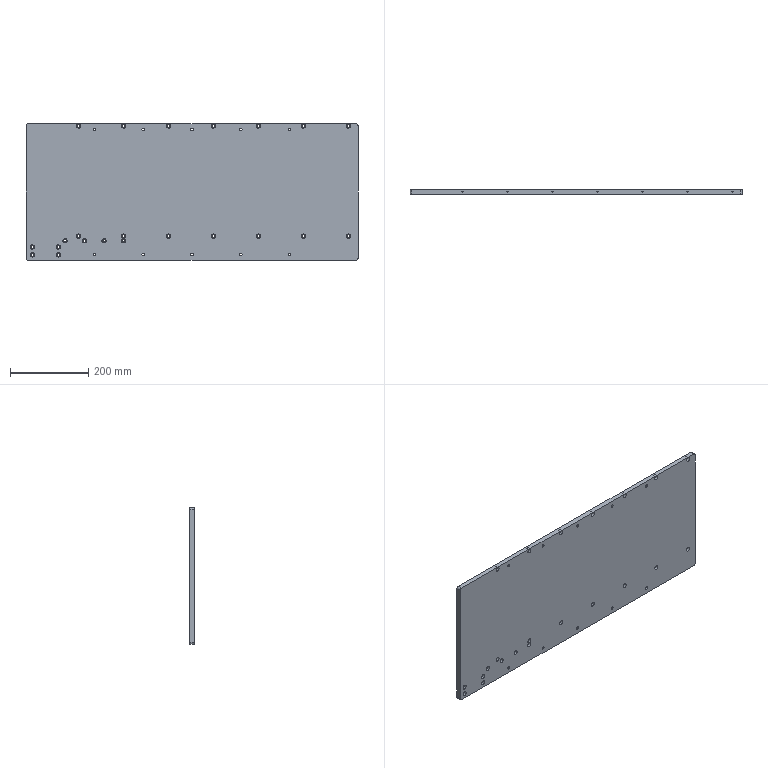Component | SolidWorks | LD101-02--Q1030-Q1-2-1 | 1 solid | 170 faces | box 850 x 12 x 350 mm | volume 3543370 mm3 | cylinder 132 | plane 38 | commonest cylinder face diameters 11 x64 6.6 x64 10 x4 | material AL6061
build123d program:
from build123d import *

# Parameters (mm, degrees)
SKETCH1_W                                          = 850
SKETCH1_H                                          = 350
BOSS_EXTRUDE1_DEPTH                                = 6
HOLE_SIZE_FOR_HEX_SOCKET_HEAD_CAP_SCRE_D           = 6.6
HOLE_SIZE_FOR_HEX_SOCKET_HEAD_CAP_SCRE_CBORE_D     = 11
HOLE_SIZE_FOR_HEX_SOCKET_HEAD_CAP_SCRE_CBORE_DEPTH = 6.8
HOLE_SIZE_FOR_HEX_SOCKET_HEAD_CAP_2_D              = 6.6
HOLE_SIZE_FOR_HEX_SOCKET_HEAD_CAP_2_CBORE_D        = 11
HOLE_SIZE_FOR_HEX_SOCKET_HEAD_CAP_2_CBORE_DEPTH    = 6.8
FILLET1_R                                          = 5
HOLE_SIZE_FOR_HEX_SOCKET_HEAD_CAP_3_D              = 6.6
HOLE_SIZE_FOR_HEX_SOCKET_HEAD_CAP_3_CBORE_D        = 11
HOLE_SIZE_FOR_HEX_SOCKET_HEAD_CAP_3_CBORE_DEPTH    = 6.8


with BuildPart() as part:
    # Sketch1 → Boss-Extrude1 (new, symmetric)
    with BuildSketch(Plane(origin=(0, 0, 0), x_dir=(1, 0, 0), z_dir=(0, 1, 0))):
        Rectangle(SKETCH1_W, SKETCH1_H)
    extrude(amount=BOSS_EXTRUDE1_DEPTH, both=True)

    # Hole Size _for_ Hex Socket Head Cap Scre (through all)
    with Locations(Plane(origin=(0, -6, 0), x_dir=(-1, 0, 0), z_dir=(0, -1, 0))):
        with Locations((175, -169), (60, -169), (-55, -169), (-170, -169), (-285, -169), (-285, 113), (-170, 113), (-55, 113), (60, 113), (175, 113), (175, 125), (225, 125), (275, 125), (325, 125), (290, 113), (290, -169), (-400, -169), (-400, 113)):
            CounterBoreHole(HOLE_SIZE_FOR_HEX_SOCKET_HEAD_CAP_SCRE_D / 2, HOLE_SIZE_FOR_HEX_SOCKET_HEAD_CAP_SCRE_CBORE_D / 2, HOLE_SIZE_FOR_HEX_SOCKET_HEAD_CAP_SCRE_CBORE_DEPTH)

    # Hole Size _for_ Hex Socket Head Cap  2 (through all)
    with Locations(Plane(origin=(0, 6, 0), x_dir=(1, 0, 0), z_dir=(0, 1, 0))):
        with Locations((-250, -160), (-125, -160), (0, -160), (250, -160), (125, -160), (250, 160), (125, 160), (0, 160), (-250, 160), (-125, 160)):
            CounterBoreHole(HOLE_SIZE_FOR_HEX_SOCKET_HEAD_CAP_2_D / 2, HOLE_SIZE_FOR_HEX_SOCKET_HEAD_CAP_2_CBORE_D / 2, HOLE_SIZE_FOR_HEX_SOCKET_HEAD_CAP_2_CBORE_DEPTH)

    # Fillet1
    fillet1_edges = [part.edges().sort_by_distance(p)[0] for p in [
        (425, 0, 175),
        (-425, 0, 175),
        (-425, 0, -175),
        (425, 0, -175),
    ]]
    fillet(fillet1_edges, radius=FILLET1_R)

    # Hole Size _for_ Hex Socket Head Cap  3 (through all)
    with Locations(Plane(origin=(0, -6, 0), x_dir=(-1, 0, 0), z_dir=(0, -1, 0))):
        with Locations((409, 161), (409, 141), (342, 161), (342, 141)):
            CounterBoreHole(HOLE_SIZE_FOR_HEX_SOCKET_HEAD_CAP_3_D / 2, HOLE_SIZE_FOR_HEX_SOCKET_HEAD_CAP_3_CBORE_D / 2, HOLE_SIZE_FOR_HEX_SOCKET_HEAD_CAP_3_CBORE_DEPTH)


solid = part.part

# Placed as in the assembly
solid = solid.moved(Location((-85.29, -245.897, 118.257), (0, 0, 0)))